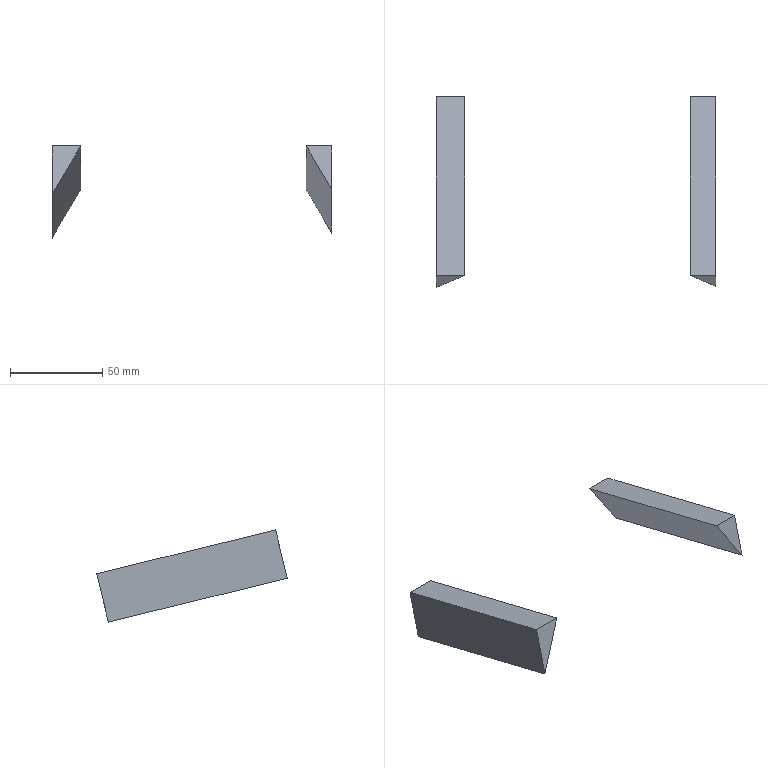Component | SolidWorks | SAV2-1 | 2 solids | 10 faces | box 152 x 103.55 x 50 mm | volume 38019 mm3 | plane 10
build123d program:
from build123d import *

# Parameters (mm, degrees)
BOSS_EXTRUDE1_DEPTH   = 100
BOSS_EXTRUDE1_2_DEPTH = 100


with BuildPart() as part:
    # Sketch2 → Boss-Extrude1 (new body)
    with BuildSketch(Plane.XY):
        Polygon((-30, 13), (-5.751, -1), (-30, -1), align=None)
    extrude(amount=-BOSS_EXTRUDE1_DEPTH)


with BuildPart() as body_2:
    # Sketch2 → Boss-Extrude1 2 (new body)
    with BuildSketch(Plane.XY):
        Polygon((-3, 151), (-30, 135.412), (-30, 151), align=None)
    extrude(amount=-BOSS_EXTRUDE1_2_DEPTH)


solid = Compound([part.part, body_2.part])

# Placed as in the assembly
solid = solid.moved(Location((0, 359.005, -132.02), (-103.755, 0, 90)))
STEP:
#1=COLOUR_RGB('',0.7922,0.8196,0.9333);
#2=FILL_AREA_STYLE_COLOUR('',#1);
#3=FILL_AREA_STYLE('',(#2));
#4=SURFACE_STYLE_FILL_AREA(#3);
#5=SURFACE_SIDE_STYLE('',(#4));
#6=SURFACE_STYLE_USAGE(.BOTH.,#5);
#7=PRESENTATION_STYLE_ASSIGNMENT((#6));
#8=CARTESIAN_POINT('',(-5.945,14.162,-5.083));
#9=VERTEX_POINT('',#8);
#10=CARTESIAN_POINT('',(-5.945,14.415,-4.05));
#11=VERTEX_POINT('',#10);
#12=CARTESIAN_POINT('',(-5.945,14.162,-5.083));
#13=DIRECTION('',(-0.,0.2378,0.9713));
#14=VECTOR('',#13,39.37);
#15=LINE('',#12,#14);
#16=EDGE_CURVE('',#9,#11,#15,.T.);
#17=ORIENTED_EDGE('',*,*,#16,.F.);
#18=CARTESIAN_POINT('',(-5.945,10.338,-4.147));
#19=VERTEX_POINT('',#18);
#20=CARTESIAN_POINT('',(-5.945,10.338,-4.147));
#21=DIRECTION('',(-0.,0.9713,-0.2378));
#22=VECTOR('',#21,39.37);
#23=LINE('',#20,#22);
#24=EDGE_CURVE('',#19,#9,#23,.T.);
#25=ORIENTED_EDGE('',*,*,#24,.F.);
#26=CARTESIAN_POINT('',(-5.945,10.591,-3.114));
#27=VERTEX_POINT('',#26);
#28=CARTESIAN_POINT('',(-5.945,10.338,-4.147));
#29=DIRECTION('',(-0.,0.2378,0.9713));
#30=VECTOR('',#29,39.37);
#31=LINE('',#28,#30);
#32=EDGE_CURVE('',#19,#27,#31,.T.);
#33=ORIENTED_EDGE('',*,*,#32,.T.);
#34=CARTESIAN_POINT('',(-5.945,10.591,-3.114));
#35=DIRECTION('',(-0.,0.9713,-0.2378));
#36=VECTOR('',#35,39.37);
#37=LINE('',#34,#36);
#38=EDGE_CURVE('',#27,#11,#37,.T.);
#39=ORIENTED_EDGE('',*,*,#38,.T.);
#40=EDGE_LOOP('',(#17,#25,#33,#39));
#41=FACE_OUTER_BOUND('',#40,.T.);
#42=CARTESIAN_POINT('',(-5.945,10.338,-4.147));
#43=DIRECTION('',(-1.,-0.,0.));
#44=DIRECTION('',(-0.,0.9713,-0.2378));
#45=AXIS2_PLACEMENT_3D('',#42,#43,#44);
#46=PLANE('',#45);
#47=ADVANCED_FACE('',(#41),#46,.T.);
#48=CARTESIAN_POINT('',(-5.331,14.415,-4.05));
#49=VERTEX_POINT('',#48);
#50=CARTESIAN_POINT('',(-5.945,14.162,-5.083));
#51=DIRECTION('',(-0.5,-0.2059,-0.8412));
#52=VECTOR('',#51,39.37);
#53=LINE('',#50,#52);
#54=EDGE_CURVE('',#49,#9,#53,.T.);
#55=ORIENTED_EDGE('',*,*,#54,.F.);
#56=CARTESIAN_POINT('',(-5.331,10.591,-3.114));
#57=VERTEX_POINT('',#56);
#58=CARTESIAN_POINT('',(-5.331,10.591,-3.114));
#59=DIRECTION('',(-0.,0.9713,-0.2378));
#60=VECTOR('',#59,39.37);
#61=LINE('',#58,#60);
#62=EDGE_CURVE('',#57,#49,#61,.T.);
#63=ORIENTED_EDGE('',*,*,#62,.F.);
#64=CARTESIAN_POINT('',(-5.945,10.338,-4.147));
#65=DIRECTION('',(-0.5,-0.2059,-0.8412));
#66=VECTOR('',#65,39.37);
#67=LINE('',#64,#66);
#68=EDGE_CURVE('',#57,#19,#67,.T.);
#69=ORIENTED_EDGE('',*,*,#68,.T.);
#70=ORIENTED_EDGE('',*,*,#24,.T.);
#71=EDGE_LOOP('',(#55,#63,#69,#70));
#72=FACE_OUTER_BOUND('',#71,.T.);
#73=CARTESIAN_POINT('',(-5.945,10.338,-4.147));
#74=DIRECTION('',(0.866,-0.1189,-0.4857));
#75=DIRECTION('',(-0.5,-0.2059,-0.8412));
#76=AXIS2_PLACEMENT_3D('',#73,#74,#75);
#77=PLANE('',#76);
#78=ADVANCED_FACE('',(#72),#77,.T.);
#79=CARTESIAN_POINT('',(-5.945,14.415,-4.05));
#80=DIRECTION('',(1.,0.,-0.));
#81=VECTOR('',#80,39.37);
#82=LINE('',#79,#81);
#83=EDGE_CURVE('',#11,#49,#82,.T.);
#84=ORIENTED_EDGE('',*,*,#83,.F.);
#85=ORIENTED_EDGE('',*,*,#38,.F.);
#86=CARTESIAN_POINT('',(-5.945,10.591,-3.114));
#87=DIRECTION('',(1.,0.,-0.));
#88=VECTOR('',#87,39.37);
#89=LINE('',#86,#88);
#90=EDGE_CURVE('',#27,#57,#89,.T.);
#91=ORIENTED_EDGE('',*,*,#90,.T.);
#92=ORIENTED_EDGE('',*,*,#62,.T.);
#93=EDGE_LOOP('',(#84,#85,#91,#92));
#94=FACE_OUTER_BOUND('',#93,.T.);
#95=CARTESIAN_POINT('',(-5.945,10.591,-3.114));
#96=DIRECTION('',(0.,0.2378,0.9713));
#97=DIRECTION('',(-0.,0.9713,-0.2378));
#98=AXIS2_PLACEMENT_3D('',#95,#96,#97);
#99=PLANE('',#98);
#100=ADVANCED_FACE('',(#94),#99,.T.);
#101=ORIENTED_EDGE('',*,*,#32,.F.);
#102=ORIENTED_EDGE('',*,*,#68,.F.);
#103=ORIENTED_EDGE('',*,*,#90,.F.);
#104=EDGE_LOOP('',(#101,#102,#103));
#105=FACE_OUTER_BOUND('',#104,.T.);
#106=CARTESIAN_POINT('',(-0.,10.31,-4.262));
#107=DIRECTION('',(-0.,0.9713,-0.2378));
#108=DIRECTION('',(0.,-0.2378,-0.9713));
#109=AXIS2_PLACEMENT_3D('',#106,#107,#108);
#110=PLANE('',#109);
#111=ADVANCED_FACE('',(#105),#110,.F.);
#112=ORIENTED_EDGE('',*,*,#16,.T.);
#113=ORIENTED_EDGE('',*,*,#83,.T.);
#114=ORIENTED_EDGE('',*,*,#54,.T.);
#115=EDGE_LOOP('',(#112,#113,#114));
#116=FACE_OUTER_BOUND('',#115,.T.);
#117=CARTESIAN_POINT('',(-0.,14.134,-5.198));
#118=DIRECTION('',(-0.,0.9713,-0.2378));
#119=DIRECTION('',(0.,-0.2378,-0.9713));
#120=AXIS2_PLACEMENT_3D('',#117,#118,#119);
#121=PLANE('',#120);
#122=ADVANCED_FACE('',(#116),#121,.T.);
#123=CLOSED_SHELL('',(#47,#78,#100,#111,#122));
#124=MANIFOLD_SOLID_BREP('',#123);
#125=STYLED_ITEM('',(#7),#124);
#126=(LENGTH_UNIT()NAMED_UNIT(*)SI_UNIT($,.METRE.));
#127=LENGTH_MEASURE_WITH_UNIT(LENGTH_MEASURE(0.0254),#126);
#128=DIMENSIONAL_EXPONENTS(1.,0.,0.,0.,0.,0.,0.);
#129=(CONVERSION_BASED_UNIT('',#127)LENGTH_UNIT()NAMED_UNIT(#128));
#130=UNCERTAINTY_MEASURE_WITH_UNIT(LENGTH_MEASURE(0.00001),#129,'','');
#131=(NAMED_UNIT(*)PLANE_ANGLE_UNIT()SI_UNIT($,.RADIAN.));
#132=(NAMED_UNIT(*)SI_UNIT($,.STERADIAN.)SOLID_ANGLE_UNIT());
#133=(GEOMETRIC_REPRESENTATION_CONTEXT(3)GLOBAL_UNCERTAINTY_ASSIGNED_CONTEXT((#130))GLOBAL_UNIT_ASSIGNED_CONTEXT((#129,#131,#132))REPRESENTATION_CONTEXT('',''));
#134=MECHANICAL_DESIGN_GEOMETRIC_PRESENTATION_REPRESENTATION('',(#125),#133);
#135=COLOUR_RGB('',0.7922,0.8196,0.9333);
#136=FILL_AREA_STYLE_COLOUR('',#135);
#137=FILL_AREA_STYLE('',(#136));
#138=SURFACE_STYLE_FILL_AREA(#137);
#139=SURFACE_SIDE_STYLE('',(#138));
#140=SURFACE_STYLE_USAGE(.BOTH.,#139);
#141=PRESENTATION_STYLE_ASSIGNMENT((#140));
#142=CARTESIAN_POINT('',(-0.5118,14.415,-4.05));
#143=VERTEX_POINT('',#142);
#144=CARTESIAN_POINT('',(0.03937,14.415,-4.05));
#145=VERTEX_POINT('',#144);
#146=CARTESIAN_POINT('',(0.03937,14.415,-4.05));
#147=DIRECTION('',(1.,-0.,-0.));
#148=VECTOR('',#147,39.37);
#149=LINE('',#146,#148);
#150=EDGE_CURVE('',#143,#145,#149,.T.);
#151=ORIENTED_EDGE('',*,*,#150,.F.);
#152=CARTESIAN_POINT('',(-0.5118,10.591,-3.114));
#153=VERTEX_POINT('',#152);
#154=CARTESIAN_POINT('',(-0.5118,10.591,-3.114));
#155=DIRECTION('',(-0.,0.9713,-0.2378));
#156=VECTOR('',#155,39.37);
#157=LINE('',#154,#156);
#158=EDGE_CURVE('',#153,#143,#157,.T.);
#159=ORIENTED_EDGE('',*,*,#158,.F.);
#160=CARTESIAN_POINT('',(0.03937,10.591,-3.114));
#161=VERTEX_POINT('',#160);
#162=CARTESIAN_POINT('',(0.03937,10.591,-3.114));
#163=DIRECTION('',(1.,-0.,-0.));
#164=VECTOR('',#163,39.37);
#165=LINE('',#162,#164);
#166=EDGE_CURVE('',#153,#161,#165,.T.);
#167=ORIENTED_EDGE('',*,*,#166,.T.);
#168=CARTESIAN_POINT('',(0.03937,10.591,-3.114));
#169=DIRECTION('',(-0.,0.9713,-0.2378));
#170=VECTOR('',#169,39.37);
#171=LINE('',#168,#170);
#172=EDGE_CURVE('',#161,#145,#171,.T.);
#173=ORIENTED_EDGE('',*,*,#172,.T.);
#174=EDGE_LOOP('',(#151,#159,#167,#173));
#175=FACE_OUTER_BOUND('',#174,.T.);
#176=CARTESIAN_POINT('',(0.03937,10.591,-3.114));
#177=DIRECTION('',(0.,0.2378,0.9713));
#178=DIRECTION('',(1.,-0.,-0.));
#179=AXIS2_PLACEMENT_3D('',#176,#177,#178);
#180=PLANE('',#179);
#181=ADVANCED_FACE('',(#175),#180,.T.);
#182=CARTESIAN_POINT('',(0.03937,14.188,-4.978));
#183=VERTEX_POINT('',#182);
#184=CARTESIAN_POINT('',(-0.5118,14.415,-4.05));
#185=DIRECTION('',(-0.5,0.2059,0.8412));
#186=VECTOR('',#185,39.37);
#187=LINE('',#184,#186);
#188=EDGE_CURVE('',#183,#143,#187,.T.);
#189=ORIENTED_EDGE('',*,*,#188,.F.);
#190=CARTESIAN_POINT('',(0.03937,10.364,-4.042));
#191=VERTEX_POINT('',#190);
#192=CARTESIAN_POINT('',(0.03937,10.364,-4.042));
#193=DIRECTION('',(-0.,0.9713,-0.2378));
#194=VECTOR('',#193,39.37);
#195=LINE('',#192,#194);
#196=EDGE_CURVE('',#191,#183,#195,.T.);
#197=ORIENTED_EDGE('',*,*,#196,.F.);
#198=CARTESIAN_POINT('',(-0.5118,10.591,-3.114));
#199=DIRECTION('',(-0.5,0.2059,0.8412));
#200=VECTOR('',#199,39.37);
#201=LINE('',#198,#200);
#202=EDGE_CURVE('',#191,#153,#201,.T.);
#203=ORIENTED_EDGE('',*,*,#202,.T.);
#204=ORIENTED_EDGE('',*,*,#158,.T.);
#205=EDGE_LOOP('',(#189,#197,#203,#204));
#206=FACE_OUTER_BOUND('',#205,.T.);
#207=CARTESIAN_POINT('',(-0.5118,10.591,-3.114));
#208=DIRECTION('',(-0.866,-0.1189,-0.4857));
#209=DIRECTION('',(-0.5,0.2059,0.8412));
#210=AXIS2_PLACEMENT_3D('',#207,#208,#209);
#211=PLANE('',#210);
#212=ADVANCED_FACE('',(#206),#211,.T.);
#213=CARTESIAN_POINT('',(0.03937,14.188,-4.978));
#214=DIRECTION('',(0.,-0.2378,-0.9713));
#215=VECTOR('',#214,39.37);
#216=LINE('',#213,#215);
#217=EDGE_CURVE('',#145,#183,#216,.T.);
#218=ORIENTED_EDGE('',*,*,#217,.F.);
#219=ORIENTED_EDGE('',*,*,#172,.F.);
#220=CARTESIAN_POINT('',(0.03937,10.364,-4.042));
#221=DIRECTION('',(0.,-0.2378,-0.9713));
#222=VECTOR('',#221,39.37);
#223=LINE('',#220,#222);
#224=EDGE_CURVE('',#161,#191,#223,.T.);
#225=ORIENTED_EDGE('',*,*,#224,.T.);
#226=ORIENTED_EDGE('',*,*,#196,.T.);
#227=EDGE_LOOP('',(#218,#219,#225,#226));
#228=FACE_OUTER_BOUND('',#227,.T.);
#229=CARTESIAN_POINT('',(0.03937,10.364,-4.042));
#230=DIRECTION('',(1.,0.,-0.));
#231=DIRECTION('',(0.,-0.2378,-0.9713));
#232=AXIS2_PLACEMENT_3D('',#229,#230,#231);
#233=PLANE('',#232);
#234=ADVANCED_FACE('',(#228),#233,.T.);
#235=ORIENTED_EDGE('',*,*,#166,.F.);
#236=ORIENTED_EDGE('',*,*,#202,.F.);
#237=ORIENTED_EDGE('',*,*,#224,.F.);
#238=EDGE_LOOP('',(#235,#236,#237));
#239=FACE_OUTER_BOUND('',#238,.T.);
#240=CARTESIAN_POINT('',(-0.,10.31,-4.262));
#241=DIRECTION('',(-0.,0.9713,-0.2378));
#242=DIRECTION('',(0.,-0.2378,-0.9713));
#243=AXIS2_PLACEMENT_3D('',#240,#241,#242);
#244=PLANE('',#243);
#245=ADVANCED_FACE('',(#239),#244,.F.);
#246=ORIENTED_EDGE('',*,*,#150,.T.);
#247=ORIENTED_EDGE('',*,*,#217,.T.);
#248=ORIENTED_EDGE('',*,*,#188,.T.);
#249=EDGE_LOOP('',(#246,#247,#248));
#250=FACE_OUTER_BOUND('',#249,.T.);
#251=CARTESIAN_POINT('',(-0.,14.134,-5.198));
#252=DIRECTION('',(-0.,0.9713,-0.2378));
#253=DIRECTION('',(0.,-0.2378,-0.9713));
#254=AXIS2_PLACEMENT_3D('',#251,#252,#253);
#255=PLANE('',#254);
#256=ADVANCED_FACE('',(#250),#255,.T.);
#257=CLOSED_SHELL('',(#181,#212,#234,#245,#256));
#258=MANIFOLD_SOLID_BREP('',#257);
#259=STYLED_ITEM('',(#141),#258);
#260=PRESENTATION_LAYER_ASSIGNMENT('','',(#259));
#261=PRESENTATION_LAYER_ASSIGNMENT('','',(#125));
#262=CARTESIAN_POINT('',(0.,0.,0.));
#263=DIRECTION('',(0.,0.,1.));
#264=DIRECTION('',(1.,0.,0.));
#265=AXIS2_PLACEMENT_3D('',#262,#263,#264);
#266=(LENGTH_UNIT()NAMED_UNIT(*)SI_UNIT($,.METRE.));
#267=LENGTH_MEASURE_WITH_UNIT(LENGTH_MEASURE(0.0254),#266);
#268=DIMENSIONAL_EXPONENTS(1.,0.,0.,0.,0.,0.,0.);
#269=(CONVERSION_BASED_UNIT('',#267)LENGTH_UNIT()NAMED_UNIT(#268));
#270=UNCERTAINTY_MEASURE_WITH_UNIT(LENGTH_MEASURE(0.00001),#269,'','');
#271=(NAMED_UNIT(*)PLANE_ANGLE_UNIT()SI_UNIT($,.RADIAN.));
#272=(NAMED_UNIT(*)SI_UNIT($,.STERADIAN.)SOLID_ANGLE_UNIT());
#273=(GEOMETRIC_REPRESENTATION_CONTEXT(3)GLOBAL_UNCERTAINTY_ASSIGNED_CONTEXT((#270))GLOBAL_UNIT_ASSIGNED_CONTEXT((#269,#271,#272))REPRESENTATION_CONTEXT('',''));
#274=ADVANCED_BREP_SHAPE_REPRESENTATION('',(#124,#258,#265),#273);
#275=(LENGTH_UNIT()NAMED_UNIT(*)SI_UNIT($,.METRE.));
#276=LENGTH_MEASURE_WITH_UNIT(LENGTH_MEASURE(0.0254),#275);
#277=DIMENSIONAL_EXPONENTS(1.,0.,0.,0.,0.,0.,0.);
#278=(CONVERSION_BASED_UNIT('',#276)LENGTH_UNIT()NAMED_UNIT(#277));
#279=UNCERTAINTY_MEASURE_WITH_UNIT(LENGTH_MEASURE(0.00001),#278,'','');
#280=(NAMED_UNIT(*)PLANE_ANGLE_UNIT()SI_UNIT($,.RADIAN.));
#281=(NAMED_UNIT(*)SI_UNIT($,.STERADIAN.)SOLID_ANGLE_UNIT());
#282=(GEOMETRIC_REPRESENTATION_CONTEXT(3)GLOBAL_UNCERTAINTY_ASSIGNED_CONTEXT((#279))GLOBAL_UNIT_ASSIGNED_CONTEXT((#278,#280,#281))REPRESENTATION_CONTEXT('',''));
#283=MECHANICAL_DESIGN_GEOMETRIC_PRESENTATION_REPRESENTATION('',(#259),#282);